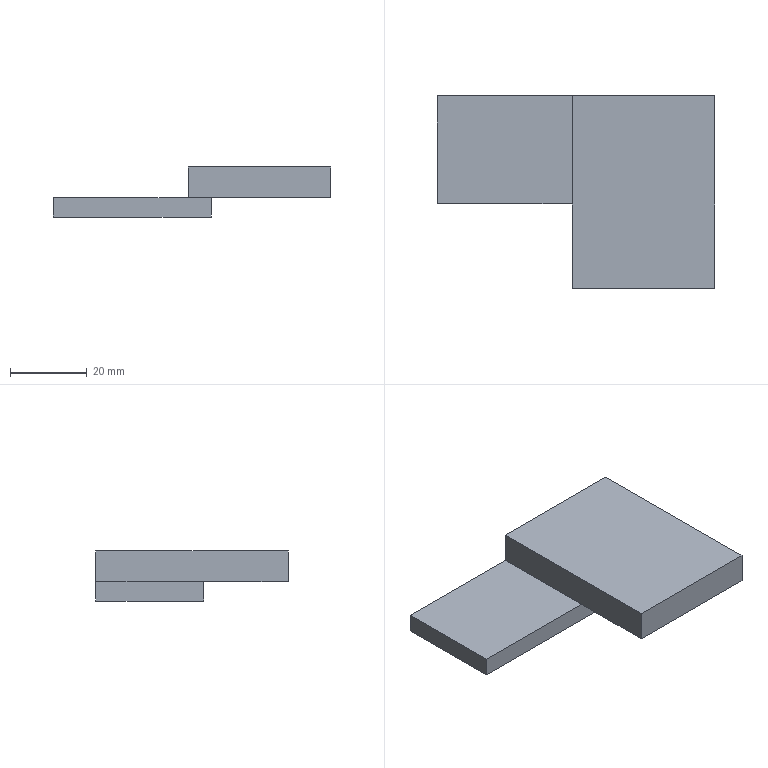Component | SolidWorks | Gripper-2024-3-4-06-1 | 1 solid | 11 faces | box 72 x 50 x 13 mm | volume 20540 mm3 | plane 11 | material S45C
STEP:
#1=COLOUR_RGB('',0.7922,0.8196,0.9333);
#2=FILL_AREA_STYLE_COLOUR('',#1);
#3=FILL_AREA_STYLE('',(#2));
#4=SURFACE_STYLE_FILL_AREA(#3);
#5=SURFACE_SIDE_STYLE('',(#4));
#6=SURFACE_STYLE_USAGE(.BOTH.,#5);
#7=PRESENTATION_STYLE_ASSIGNMENT((#6));
#8=CARTESIAN_POINT('',(-6.049,-0.2685,10.276));
#9=VERTEX_POINT('',#8);
#10=CARTESIAN_POINT('',(-6.049,-1.371,10.276));
#11=VERTEX_POINT('',#10);
#12=CARTESIAN_POINT('',(-6.049,-0.2685,10.276));
#13=DIRECTION('',(-0.,-1.,0.));
#14=VECTOR('',#13,39.37);
#15=LINE('',#12,#14);
#16=EDGE_CURVE('',#9,#11,#15,.T.);
#17=ORIENTED_EDGE('',*,*,#16,.T.);
#18=CARTESIAN_POINT('',(-6.049,-1.371,10.472));
#19=VERTEX_POINT('',#18);
#20=CARTESIAN_POINT('',(-6.049,-1.371,11.85));
#21=DIRECTION('',(0.,-0.,-1.));
#22=VECTOR('',#21,39.37);
#23=LINE('',#20,#22);
#24=EDGE_CURVE('',#19,#11,#23,.T.);
#25=ORIENTED_EDGE('',*,*,#24,.F.);
#26=CARTESIAN_POINT('',(-6.049,-0.2685,10.472));
#27=VERTEX_POINT('',#26);
#28=CARTESIAN_POINT('',(-6.049,-0.2685,10.472));
#29=DIRECTION('',(-0.,-1.,0.));
#30=VECTOR('',#29,39.37);
#31=LINE('',#28,#30);
#32=EDGE_CURVE('',#27,#19,#31,.T.);
#33=ORIENTED_EDGE('',*,*,#32,.F.);
#34=CARTESIAN_POINT('',(-6.049,-0.2685,10.472));
#35=DIRECTION('',(-0.,0.,1.));
#36=VECTOR('',#35,39.37);
#37=LINE('',#34,#36);
#38=EDGE_CURVE('',#9,#27,#37,.T.);
#39=ORIENTED_EDGE('',*,*,#38,.F.);
#40=EDGE_LOOP('',(#17,#25,#33,#39));
#41=FACE_OUTER_BOUND('',#40,.T.);
#42=CARTESIAN_POINT('',(-6.049,-0.2685,10.472));
#43=DIRECTION('',(1.,-0.,0.));
#44=DIRECTION('',(-0.,-1.,0.));
#45=AXIS2_PLACEMENT_3D('',#42,#43,#44);
#46=PLANE('',#45);
#47=ADVANCED_FACE('',(#41),#46,.F.);
#48=ORIENTED_EDGE('',*,*,#32,.T.);
#49=CARTESIAN_POINT('',(-4.671,-1.371,10.472));
#50=VERTEX_POINT('',#49);
#51=CARTESIAN_POINT('',(-6.049,-1.371,10.472));
#52=DIRECTION('',(1.,-0.,0.));
#53=VECTOR('',#52,39.37);
#54=LINE('',#51,#53);
#55=EDGE_CURVE('',#19,#50,#54,.T.);
#56=ORIENTED_EDGE('',*,*,#55,.T.);
#57=CARTESIAN_POINT('',(-4.671,-0.2685,10.472));
#58=VERTEX_POINT('',#57);
#59=CARTESIAN_POINT('',(-4.671,-0.2685,10.472));
#60=DIRECTION('',(-0.,-1.,0.));
#61=VECTOR('',#60,39.37);
#62=LINE('',#59,#61);
#63=EDGE_CURVE('',#58,#50,#62,.T.);
#64=ORIENTED_EDGE('',*,*,#63,.F.);
#65=CARTESIAN_POINT('',(-6.049,-0.2685,10.472));
#66=DIRECTION('',(1.,-0.,0.));
#67=VECTOR('',#66,39.37);
#68=LINE('',#65,#67);
#69=EDGE_CURVE('',#27,#58,#68,.T.);
#70=ORIENTED_EDGE('',*,*,#69,.F.);
#71=EDGE_LOOP('',(#48,#56,#64,#70));
#72=FACE_OUTER_BOUND('',#71,.T.);
#73=CARTESIAN_POINT('',(-6.049,-0.2685,10.472));
#74=DIRECTION('',(0.,-0.,-1.));
#75=DIRECTION('',(0.,1.,-0.));
#76=AXIS2_PLACEMENT_3D('',#73,#74,#75);
#77=PLANE('',#76);
#78=ADVANCED_FACE('',(#72),#77,.F.);
#79=ORIENTED_EDGE('',*,*,#63,.T.);
#80=CARTESIAN_POINT('',(-4.671,-2.237,10.472));
#81=VERTEX_POINT('',#80);
#82=CARTESIAN_POINT('',(-4.671,-0.2685,10.472));
#83=DIRECTION('',(-0.,-1.,0.));
#84=VECTOR('',#83,39.37);
#85=LINE('',#82,#84);
#86=EDGE_CURVE('',#50,#81,#85,.T.);
#87=ORIENTED_EDGE('',*,*,#86,.T.);
#88=CARTESIAN_POINT('',(-4.671,-2.237,10.787));
#89=VERTEX_POINT('',#88);
#90=CARTESIAN_POINT('',(-4.671,-2.237,10.472));
#91=DIRECTION('',(-0.,0.,1.));
#92=VECTOR('',#91,39.37);
#93=LINE('',#90,#92);
#94=EDGE_CURVE('',#81,#89,#93,.T.);
#95=ORIENTED_EDGE('',*,*,#94,.T.);
#96=CARTESIAN_POINT('',(-4.671,-0.2685,10.787));
#97=VERTEX_POINT('',#96);
#98=CARTESIAN_POINT('',(-4.671,-0.2685,10.787));
#99=DIRECTION('',(-0.,-1.,0.));
#100=VECTOR('',#99,39.37);
#101=LINE('',#98,#100);
#102=EDGE_CURVE('',#97,#89,#101,.T.);
#103=ORIENTED_EDGE('',*,*,#102,.F.);
#104=CARTESIAN_POINT('',(-4.671,-0.2685,10.472));
#105=DIRECTION('',(-0.,0.,1.));
#106=VECTOR('',#105,39.37);
#107=LINE('',#104,#106);
#108=EDGE_CURVE('',#58,#97,#107,.T.);
#109=ORIENTED_EDGE('',*,*,#108,.F.);
#110=EDGE_LOOP('',(#79,#87,#95,#103,#109));
#111=FACE_OUTER_BOUND('',#110,.T.);
#112=CARTESIAN_POINT('',(-4.671,-0.2685,10.472));
#113=DIRECTION('',(1.,-0.,0.));
#114=DIRECTION('',(-0.,-1.,0.));
#115=AXIS2_PLACEMENT_3D('',#112,#113,#114);
#116=PLANE('',#115);
#117=ADVANCED_FACE('',(#111),#116,.F.);
#118=CARTESIAN_POINT('',(-3.215,-2.237,10.787));
#119=VERTEX_POINT('',#118);
#120=CARTESIAN_POINT('',(-4.671,-2.237,10.787));
#121=DIRECTION('',(1.,-0.,0.));
#122=VECTOR('',#121,39.37);
#123=LINE('',#120,#122);
#124=EDGE_CURVE('',#89,#119,#123,.T.);
#125=ORIENTED_EDGE('',*,*,#124,.T.);
#126=CARTESIAN_POINT('',(-3.215,-0.2685,10.787));
#127=VERTEX_POINT('',#126);
#128=CARTESIAN_POINT('',(-3.215,-0.2685,10.787));
#129=DIRECTION('',(-0.,-1.,0.));
#130=VECTOR('',#129,39.37);
#131=LINE('',#128,#130);
#132=EDGE_CURVE('',#127,#119,#131,.T.);
#133=ORIENTED_EDGE('',*,*,#132,.F.);
#134=CARTESIAN_POINT('',(-4.671,-0.2685,10.787));
#135=DIRECTION('',(1.,-0.,0.));
#136=VECTOR('',#135,39.37);
#137=LINE('',#134,#136);
#138=EDGE_CURVE('',#97,#127,#137,.T.);
#139=ORIENTED_EDGE('',*,*,#138,.F.);
#140=ORIENTED_EDGE('',*,*,#102,.T.);
#141=EDGE_LOOP('',(#125,#133,#139,#140));
#142=FACE_OUTER_BOUND('',#141,.T.);
#143=CARTESIAN_POINT('',(-4.671,-0.2685,10.787));
#144=DIRECTION('',(0.,-0.,-1.));
#145=DIRECTION('',(0.,1.,-0.));
#146=AXIS2_PLACEMENT_3D('',#143,#144,#145);
#147=PLANE('',#146);
#148=ADVANCED_FACE('',(#142),#147,.F.);
#149=CARTESIAN_POINT('',(-3.215,-2.237,10.472));
#150=VERTEX_POINT('',#149);
#151=CARTESIAN_POINT('',(-3.215,-2.237,10.472));
#152=DIRECTION('',(0.,-0.,-1.));
#153=VECTOR('',#152,39.37);
#154=LINE('',#151,#153);
#155=EDGE_CURVE('',#119,#150,#154,.T.);
#156=ORIENTED_EDGE('',*,*,#155,.T.);
#157=CARTESIAN_POINT('',(-3.215,-0.2685,10.472));
#158=VERTEX_POINT('',#157);
#159=CARTESIAN_POINT('',(-3.215,-0.2685,10.472));
#160=DIRECTION('',(-0.,-1.,0.));
#161=VECTOR('',#160,39.37);
#162=LINE('',#159,#161);
#163=EDGE_CURVE('',#158,#150,#162,.T.);
#164=ORIENTED_EDGE('',*,*,#163,.F.);
#165=CARTESIAN_POINT('',(-3.215,-0.2685,10.472));
#166=DIRECTION('',(0.,-0.,-1.));
#167=VECTOR('',#166,39.37);
#168=LINE('',#165,#167);
#169=EDGE_CURVE('',#127,#158,#168,.T.);
#170=ORIENTED_EDGE('',*,*,#169,.F.);
#171=ORIENTED_EDGE('',*,*,#132,.T.);
#172=EDGE_LOOP('',(#156,#164,#170,#171));
#173=FACE_OUTER_BOUND('',#172,.T.);
#174=CARTESIAN_POINT('',(-3.215,-0.2685,10.472));
#175=DIRECTION('',(-1.,0.,-0.));
#176=DIRECTION('',(0.,1.,-0.));
#177=AXIS2_PLACEMENT_3D('',#174,#175,#176);
#178=PLANE('',#177);
#179=ADVANCED_FACE('',(#173),#178,.F.);
#180=CARTESIAN_POINT('',(-4.435,-2.237,10.472));
#181=DIRECTION('',(-1.,0.,-0.));
#182=VECTOR('',#181,39.37);
#183=LINE('',#180,#182);
#184=EDGE_CURVE('',#150,#81,#183,.T.);
#185=ORIENTED_EDGE('',*,*,#184,.T.);
#186=ORIENTED_EDGE('',*,*,#86,.F.);
#187=CARTESIAN_POINT('',(-4.435,-1.371,10.472));
#188=VERTEX_POINT('',#187);
#189=CARTESIAN_POINT('',(-6.01,-1.371,10.472));
#190=DIRECTION('',(1.,-0.,0.));
#191=VECTOR('',#190,39.37);
#192=LINE('',#189,#191);
#193=EDGE_CURVE('',#50,#188,#192,.T.);
#194=ORIENTED_EDGE('',*,*,#193,.T.);
#195=CARTESIAN_POINT('',(-4.435,-0.2685,10.472));
#196=VERTEX_POINT('',#195);
#197=CARTESIAN_POINT('',(-4.435,-0.2685,10.472));
#198=DIRECTION('',(-0.,-1.,0.));
#199=VECTOR('',#198,39.37);
#200=LINE('',#197,#199);
#201=EDGE_CURVE('',#196,#188,#200,.T.);
#202=ORIENTED_EDGE('',*,*,#201,.F.);
#203=CARTESIAN_POINT('',(-4.435,-0.2685,10.472));
#204=DIRECTION('',(-1.,0.,-0.));
#205=VECTOR('',#204,39.37);
#206=LINE('',#203,#205);
#207=EDGE_CURVE('',#158,#196,#206,.T.);
#208=ORIENTED_EDGE('',*,*,#207,.F.);
#209=ORIENTED_EDGE('',*,*,#163,.T.);
#210=EDGE_LOOP('',(#185,#186,#194,#202,#208,#209));
#211=FACE_OUTER_BOUND('',#210,.T.);
#212=CARTESIAN_POINT('',(-4.435,-0.2685,10.472));
#213=DIRECTION('',(-0.,0.,1.));
#214=DIRECTION('',(-0.,-1.,0.));
#215=AXIS2_PLACEMENT_3D('',#212,#213,#214);
#216=PLANE('',#215);
#217=ADVANCED_FACE('',(#211),#216,.F.);
#218=ORIENTED_EDGE('',*,*,#201,.T.);
#219=CARTESIAN_POINT('',(-4.435,-1.371,10.276));
#220=VERTEX_POINT('',#219);
#221=CARTESIAN_POINT('',(-4.435,-1.371,10.276));
#222=DIRECTION('',(0.,0.,1.));
#223=VECTOR('',#222,39.37);
#224=LINE('',#221,#223);
#225=EDGE_CURVE('',#220,#188,#224,.T.);
#226=ORIENTED_EDGE('',*,*,#225,.F.);
#227=CARTESIAN_POINT('',(-4.435,-0.2685,10.276));
#228=VERTEX_POINT('',#227);
#229=CARTESIAN_POINT('',(-4.435,-0.2685,10.276));
#230=DIRECTION('',(-0.,-1.,0.));
#231=VECTOR('',#230,39.37);
#232=LINE('',#229,#231);
#233=EDGE_CURVE('',#228,#220,#232,.T.);
#234=ORIENTED_EDGE('',*,*,#233,.F.);
#235=CARTESIAN_POINT('',(-4.435,-0.2685,10.472));
#236=DIRECTION('',(0.,-0.,-1.));
#237=VECTOR('',#236,39.37);
#238=LINE('',#235,#237);
#239=EDGE_CURVE('',#196,#228,#238,.T.);
#240=ORIENTED_EDGE('',*,*,#239,.F.);
#241=EDGE_LOOP('',(#218,#226,#234,#240));
#242=FACE_OUTER_BOUND('',#241,.T.);
#243=CARTESIAN_POINT('',(-4.435,-0.2685,10.472));
#244=DIRECTION('',(-1.,0.,-0.));
#245=DIRECTION('',(0.,1.,-0.));
#246=AXIS2_PLACEMENT_3D('',#243,#244,#245);
#247=PLANE('',#246);
#248=ADVANCED_FACE('',(#242),#247,.F.);
#249=ORIENTED_EDGE('',*,*,#233,.T.);
#250=CARTESIAN_POINT('',(-6.049,-1.371,10.276));
#251=DIRECTION('',(1.,-0.,0.));
#252=VECTOR('',#251,39.37);
#253=LINE('',#250,#252);
#254=EDGE_CURVE('',#11,#220,#253,.T.);
#255=ORIENTED_EDGE('',*,*,#254,.F.);
#256=ORIENTED_EDGE('',*,*,#16,.F.);
#257=CARTESIAN_POINT('',(-6.049,-0.2685,10.276));
#258=DIRECTION('',(-1.,0.,-0.));
#259=VECTOR('',#258,39.37);
#260=LINE('',#257,#259);
#261=EDGE_CURVE('',#228,#9,#260,.T.);
#262=ORIENTED_EDGE('',*,*,#261,.F.);
#263=EDGE_LOOP('',(#249,#255,#256,#262));
#264=FACE_OUTER_BOUND('',#263,.T.);
#265=CARTESIAN_POINT('',(-6.049,-0.2685,10.276));
#266=DIRECTION('',(-0.,0.,1.));
#267=DIRECTION('',(-0.,-1.,0.));
#268=AXIS2_PLACEMENT_3D('',#265,#266,#267);
#269=PLANE('',#268);
#270=ADVANCED_FACE('',(#264),#269,.F.);
#271=ORIENTED_EDGE('',*,*,#38,.T.);
#272=ORIENTED_EDGE('',*,*,#69,.T.);
#273=ORIENTED_EDGE('',*,*,#108,.T.);
#274=ORIENTED_EDGE('',*,*,#138,.T.);
#275=ORIENTED_EDGE('',*,*,#169,.T.);
#276=ORIENTED_EDGE('',*,*,#207,.T.);
#277=ORIENTED_EDGE('',*,*,#239,.T.);
#278=ORIENTED_EDGE('',*,*,#261,.T.);
#279=EDGE_LOOP('',(#271,#272,#273,#274,#275,#276,#277,#278));
#280=FACE_OUTER_BOUND('',#279,.T.);
#281=CARTESIAN_POINT('',(-6.049,-0.2685,10.472));
#282=DIRECTION('',(-0.,-1.,0.));
#283=DIRECTION('',(-1.,0.,-0.));
#284=AXIS2_PLACEMENT_3D('',#281,#282,#283);
#285=PLANE('',#284);
#286=ADVANCED_FACE('',(#280),#285,.F.);
#287=ORIENTED_EDGE('',*,*,#94,.F.);
#288=ORIENTED_EDGE('',*,*,#184,.F.);
#289=ORIENTED_EDGE('',*,*,#155,.F.);
#290=ORIENTED_EDGE('',*,*,#124,.F.);
#291=EDGE_LOOP('',(#287,#288,#289,#290));
#292=FACE_OUTER_BOUND('',#291,.T.);
#293=CARTESIAN_POINT('',(-6.049,-2.237,10.472));
#294=DIRECTION('',(-0.,-1.,0.));
#295=DIRECTION('',(-1.,0.,-0.));
#296=AXIS2_PLACEMENT_3D('',#293,#294,#295);
#297=PLANE('',#296);
#298=ADVANCED_FACE('',(#292),#297,.T.);
#299=ORIENTED_EDGE('',*,*,#193,.F.);
#300=ORIENTED_EDGE('',*,*,#55,.F.);
#301=ORIENTED_EDGE('',*,*,#24,.T.);
#302=ORIENTED_EDGE('',*,*,#254,.T.);
#303=ORIENTED_EDGE('',*,*,#225,.T.);
#304=EDGE_LOOP('',(#299,#300,#301,#302,#303));
#305=FACE_OUTER_BOUND('',#304,.T.);
#306=CARTESIAN_POINT('',(-6.049,-1.371,11.85));
#307=DIRECTION('',(0.,1.,-0.));
#308=DIRECTION('',(1.,-0.,0.));
#309=AXIS2_PLACEMENT_3D('',#306,#307,#308);
#310=PLANE('',#309);
#311=ADVANCED_FACE('',(#305),#310,.F.);
#312=CLOSED_SHELL('',(#47,#78,#117,#148,#179,#217,#248,#270,#286,#298,#311));
#313=MANIFOLD_SOLID_BREP('',#312);
#314=STYLED_ITEM('',(#7),#313);
#315=PRESENTATION_LAYER_ASSIGNMENT('','',(#314));
#316=(LENGTH_UNIT()NAMED_UNIT(*)SI_UNIT($,.METRE.));
#317=LENGTH_MEASURE_WITH_UNIT(LENGTH_MEASURE(0.0254),#316);
#318=DIMENSIONAL_EXPONENTS(1.,0.,0.,0.,0.,0.,0.);
#319=(CONVERSION_BASED_UNIT('',#317)LENGTH_UNIT()NAMED_UNIT(#318));
#320=UNCERTAINTY_MEASURE_WITH_UNIT(LENGTH_MEASURE(0.00001),#319,'','');
#321=(NAMED_UNIT(*)PLANE_ANGLE_UNIT()SI_UNIT($,.RADIAN.));
#322=(NAMED_UNIT(*)SI_UNIT($,.STERADIAN.)SOLID_ANGLE_UNIT());
#323=(GEOMETRIC_REPRESENTATION_CONTEXT(3)GLOBAL_UNCERTAINTY_ASSIGNED_CONTEXT((#320))GLOBAL_UNIT_ASSIGNED_CONTEXT((#319,#321,#322))REPRESENTATION_CONTEXT('',''));
#324=MECHANICAL_DESIGN_GEOMETRIC_PRESENTATION_REPRESENTATION('',(#314),#323);
#325=CARTESIAN_POINT('',(0.,0.,0.));
#326=DIRECTION('',(0.,0.,1.));
#327=DIRECTION('',(1.,0.,0.));
#328=AXIS2_PLACEMENT_3D('',#325,#326,#327);
#329=(LENGTH_UNIT()NAMED_UNIT(*)SI_UNIT($,.METRE.));
#330=LENGTH_MEASURE_WITH_UNIT(LENGTH_MEASURE(0.0254),#329);
#331=DIMENSIONAL_EXPONENTS(1.,0.,0.,0.,0.,0.,0.);
#332=(CONVERSION_BASED_UNIT('',#330)LENGTH_UNIT()NAMED_UNIT(#331));
#333=UNCERTAINTY_MEASURE_WITH_UNIT(LENGTH_MEASURE(0.00001),#332,'','');
#334=(NAMED_UNIT(*)PLANE_ANGLE_UNIT()SI_UNIT($,.RADIAN.));
#335=(NAMED_UNIT(*)SI_UNIT($,.STERADIAN.)SOLID_ANGLE_UNIT());
#336=(GEOMETRIC_REPRESENTATION_CONTEXT(3)GLOBAL_UNCERTAINTY_ASSIGNED_CONTEXT((#333))GLOBAL_UNIT_ASSIGNED_CONTEXT((#332,#334,#335))REPRESENTATION_CONTEXT('',''));
#337=ADVANCED_BREP_SHAPE_REPRESENTATION('',(#313,#328),#336);